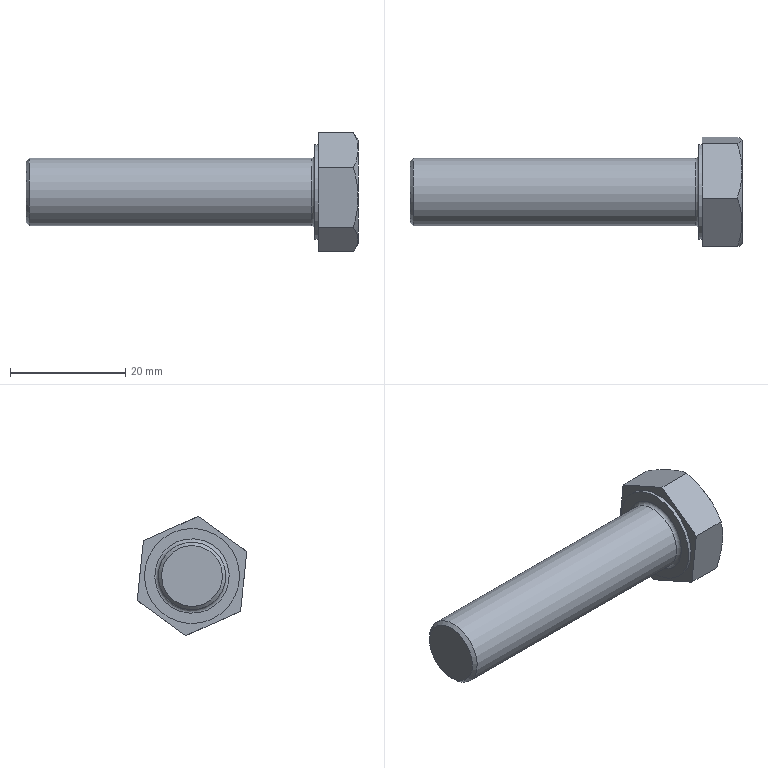Component | NX | GB-T5782-2000_M12X50 | 1 solid | 20 faces | volume 7431 mm3 | plane 10 | cone 7 | cylinder 2 | torus 1 | commonest cylinder face diameters 16.47 x1 11.701 x1